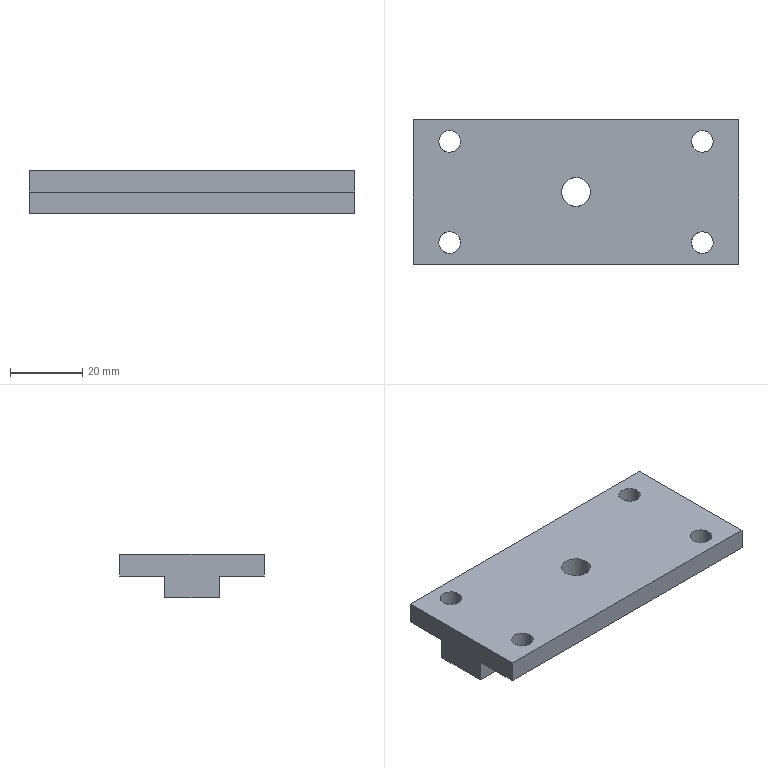Component | NX | UPPER_COVER | 1 solid | 15 faces | volume 28418 mm3 | plane 10 | cylinder 5 | commonest cylinder face diameters 6 x4 8 x1